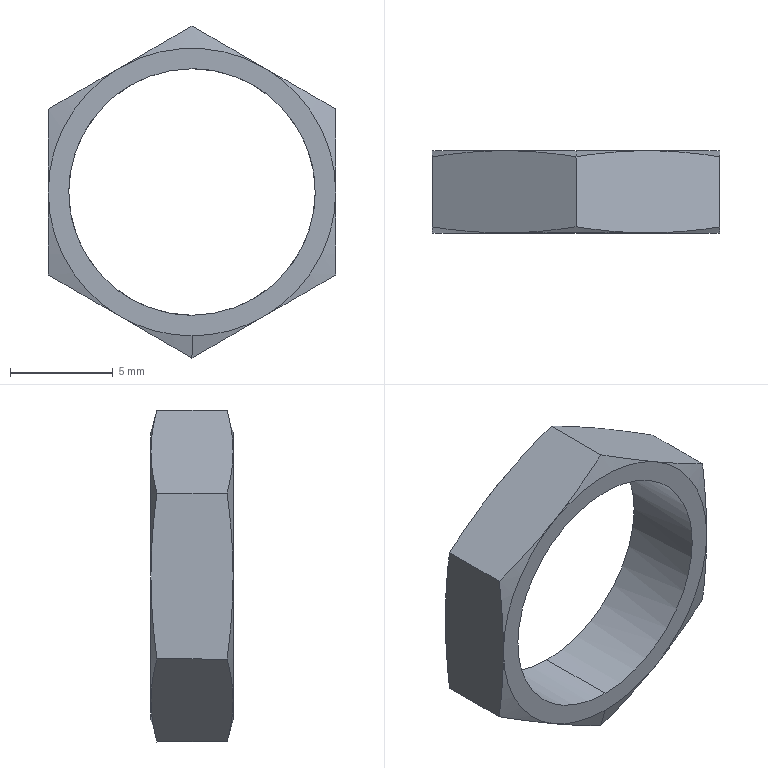Component | SolidWorks | HandlingMechanism-2_MVPTN2-1_4_1-1 | 1 solid | 24 faces | box 14 x 4 x 16.17 mm | volume 224 mm3 | cone 14 | plane 8 | cylinder 2 | commonest cylinder face diameters 12 x2
STEP:
#1=COLOUR_RGB('',0.7922,0.8196,0.9333);
#2=FILL_AREA_STYLE_COLOUR('',#1);
#3=FILL_AREA_STYLE('',(#2));
#4=SURFACE_STYLE_FILL_AREA(#3);
#5=SURFACE_SIDE_STYLE('',(#4));
#6=SURFACE_STYLE_USAGE(.BOTH.,#5);
#7=PRESENTATION_STYLE_ASSIGNMENT((#6));
#8=CARTESIAN_POINT('',(1.019,8.76,5.236));
#9=VERTEX_POINT('',#8);
#10=CARTESIAN_POINT('',(1.019,8.76,5.709));
#11=VERTEX_POINT('',#10);
#12=CARTESIAN_POINT('',(1.019,8.76,5.472));
#13=DIRECTION('',(-0.,-1.,0.));
#14=DIRECTION('',(0.,0.,1.));
#15=AXIS2_PLACEMENT_3D('',#12,#13,#14);
#16=CIRCLE('',#15,0.2362);
#17=EDGE_CURVE('',#9,#11,#16,.T.);
#18=ORIENTED_EDGE('',*,*,#17,.F.);
#19=CARTESIAN_POINT('',(1.019,8.602,5.236));
#20=VERTEX_POINT('',#19);
#21=CARTESIAN_POINT('',(1.019,8.76,5.236));
#22=DIRECTION('',(-0.,-1.,0.));
#23=VECTOR('',#22,39.37);
#24=LINE('',#21,#23);
#25=EDGE_CURVE('',#9,#20,#24,.T.);
#26=ORIENTED_EDGE('',*,*,#25,.T.);
#27=CARTESIAN_POINT('',(1.019,8.602,5.709));
#28=VERTEX_POINT('',#27);
#29=CARTESIAN_POINT('',(1.019,8.602,5.236));
#30=CARTESIAN_POINT('',(1.05,8.602,5.236));
#31=CARTESIAN_POINT('',(1.081,8.602,5.242));
#32=CARTESIAN_POINT('',(1.138,8.602,5.266));
#33=CARTESIAN_POINT('',(1.164,8.602,5.284));
#34=CARTESIAN_POINT('',(1.208,8.602,5.327));
#35=CARTESIAN_POINT('',(1.225,8.602,5.353));
#36=CARTESIAN_POINT('',(1.249,8.602,5.411));
#37=CARTESIAN_POINT('',(1.255,8.602,5.442));
#38=CARTESIAN_POINT('',(1.255,8.602,5.503));
#39=CARTESIAN_POINT('',(1.249,8.602,5.534));
#40=CARTESIAN_POINT('',(1.225,8.602,5.591));
#41=CARTESIAN_POINT('',(1.208,8.602,5.618));
#42=CARTESIAN_POINT('',(1.164,8.602,5.661));
#43=CARTESIAN_POINT('',(1.138,8.602,5.679));
#44=CARTESIAN_POINT('',(1.081,8.602,5.703));
#45=CARTESIAN_POINT('',(1.05,8.602,5.709));
#46=CARTESIAN_POINT('',(1.019,8.602,5.709));
#47=B_SPLINE_CURVE_WITH_KNOTS('',3,(#29,#30,#31,#32,#33,#34,#35,#36,#37,#38,#39,#40,#41,#42,#43,#44,#45,#46),.UNSPECIFIED.,.F.,.F.,(4,2,2,2,2,2,2,2,4),(0.5,0.5625,0.625,0.6875,0.75,0.8125,0.875,0.9375,1.),.UNSPECIFIED.);
#48=EDGE_CURVE('',#20,#28,#47,.T.);
#49=ORIENTED_EDGE('',*,*,#48,.T.);
#50=CARTESIAN_POINT('',(1.019,8.76,5.709));
#51=DIRECTION('',(-0.,-1.,0.));
#52=VECTOR('',#51,39.37);
#53=LINE('',#50,#52);
#54=EDGE_CURVE('',#11,#28,#53,.T.);
#55=ORIENTED_EDGE('',*,*,#54,.F.);
#56=EDGE_LOOP('',(#18,#26,#49,#55));
#57=FACE_OUTER_BOUND('',#56,.T.);
#58=CARTESIAN_POINT('',(1.019,8.76,5.472));
#59=DIRECTION('',(-0.,-1.,0.));
#60=DIRECTION('',(0.,0.,1.));
#61=AXIS2_PLACEMENT_3D('',#58,#59,#60);
#62=CYLINDRICAL_SURFACE('',#61,0.2362);
#63=ADVANCED_FACE('',(#57),#62,.F.);
#64=CARTESIAN_POINT('',(1.019,8.76,5.748));
#65=VERTEX_POINT('',#64);
#66=CARTESIAN_POINT('',(1.157,8.76,5.711));
#67=VERTEX_POINT('',#66);
#68=CARTESIAN_POINT('',(1.019,8.76,5.472));
#69=DIRECTION('',(0.,1.,-0.));
#70=DIRECTION('',(0.,0.,1.));
#71=AXIS2_PLACEMENT_3D('',#68,#69,#70);
#72=CIRCLE('',#71,0.2756);
#73=EDGE_CURVE('',#65,#67,#72,.T.);
#74=ORIENTED_EDGE('',*,*,#73,.F.);
#75=CARTESIAN_POINT('',(1.019,8.748,5.791));
#76=VERTEX_POINT('',#75);
#77=CARTESIAN_POINT('',(1.019,8.748,5.791));
#78=DIRECTION('',(-0.,-0.2588,0.9659));
#79=VECTOR('',#78,39.37);
#80=LINE('',#77,#79);
#81=EDGE_CURVE('',#65,#76,#80,.T.);
#82=ORIENTED_EDGE('',*,*,#81,.T.);
#83=CARTESIAN_POINT('',(1.019,8.748,5.791));
#84=CARTESIAN_POINT('',(1.065,8.755,5.764));
#85=CARTESIAN_POINT('',(1.111,8.76,5.738));
#86=CARTESIAN_POINT('',(1.157,8.76,5.711));
#87=B_SPLINE_CURVE_WITH_KNOTS('',3,(#83,#84,#85,#86),.UNSPECIFIED.,.F.,.F.,(4,4),(0.,0.004052),.UNSPECIFIED.);
#88=EDGE_CURVE('',#76,#67,#87,.T.);
#89=ORIENTED_EDGE('',*,*,#88,.T.);
#90=EDGE_LOOP('',(#74,#82,#89));
#91=FACE_OUTER_BOUND('',#90,.T.);
#92=CARTESIAN_POINT('',(1.019,8.748,5.472));
#93=DIRECTION('',(-0.,-1.,0.));
#94=DIRECTION('',(0.,0.,1.));
#95=AXIS2_PLACEMENT_3D('',#92,#93,#94);
#96=CONICAL_SURFACE('',#95,0.3185,1.309);
#97=ADVANCED_FACE('',(#91),#96,.T.);
#98=CARTESIAN_POINT('',(1.019,8.602,5.197));
#99=VERTEX_POINT('',#98);
#100=CARTESIAN_POINT('',(1.157,8.602,5.234));
#101=VERTEX_POINT('',#100);
#102=CARTESIAN_POINT('',(1.019,8.602,5.472));
#103=DIRECTION('',(-0.,-1.,0.));
#104=DIRECTION('',(0.,0.,-1.));
#105=AXIS2_PLACEMENT_3D('',#102,#103,#104);
#106=CIRCLE('',#105,0.2756);
#107=EDGE_CURVE('',#99,#101,#106,.T.);
#108=ORIENTED_EDGE('',*,*,#107,.F.);
#109=CARTESIAN_POINT('',(1.019,8.614,5.154));
#110=VERTEX_POINT('',#109);
#111=CARTESIAN_POINT('',(1.019,8.614,5.154));
#112=DIRECTION('',(0.,0.2588,-0.9659));
#113=VECTOR('',#112,39.37);
#114=LINE('',#111,#113);
#115=EDGE_CURVE('',#99,#110,#114,.T.);
#116=ORIENTED_EDGE('',*,*,#115,.T.);
#117=CARTESIAN_POINT('',(1.019,8.614,5.154));
#118=CARTESIAN_POINT('',(1.065,8.607,5.181));
#119=CARTESIAN_POINT('',(1.111,8.602,5.207));
#120=CARTESIAN_POINT('',(1.157,8.602,5.234));
#121=B_SPLINE_CURVE_WITH_KNOTS('',3,(#117,#118,#119,#120),.UNSPECIFIED.,.F.,.F.,(4,4),(0.,0.004052),.UNSPECIFIED.);
#122=EDGE_CURVE('',#110,#101,#121,.T.);
#123=ORIENTED_EDGE('',*,*,#122,.T.);
#124=EDGE_LOOP('',(#108,#116,#123));
#125=FACE_OUTER_BOUND('',#124,.T.);
#126=CARTESIAN_POINT('',(1.019,8.614,5.472));
#127=DIRECTION('',(0.,1.,-0.));
#128=DIRECTION('',(0.,0.,-1.));
#129=AXIS2_PLACEMENT_3D('',#126,#127,#128);
#130=CONICAL_SURFACE('',#129,0.3185,1.309);
#131=ADVANCED_FACE('',(#125),#130,.T.);
#132=CARTESIAN_POINT('',(1.157,8.76,5.234));
#133=VERTEX_POINT('',#132);
#134=CARTESIAN_POINT('',(0.8811,8.76,5.234));
#135=VERTEX_POINT('',#134);
#136=CARTESIAN_POINT('',(1.019,8.76,5.472));
#137=DIRECTION('',(0.,1.,-0.));
#138=DIRECTION('',(-0.,0.,1.));
#139=AXIS2_PLACEMENT_3D('',#136,#137,#138);
#140=CIRCLE('',#139,0.2756);
#141=EDGE_CURVE('',#133,#135,#140,.T.);
#142=ORIENTED_EDGE('',*,*,#141,.T.);
#143=CARTESIAN_POINT('',(0.7433,8.76,5.472));
#144=VERTEX_POINT('',#143);
#145=CARTESIAN_POINT('',(1.019,8.76,5.472));
#146=DIRECTION('',(0.,1.,-0.));
#147=DIRECTION('',(0.,0.,1.));
#148=AXIS2_PLACEMENT_3D('',#145,#146,#147);
#149=CIRCLE('',#148,0.2756);
#150=EDGE_CURVE('',#135,#144,#149,.T.);
#151=ORIENTED_EDGE('',*,*,#150,.T.);
#152=CARTESIAN_POINT('',(0.8811,8.76,5.711));
#153=VERTEX_POINT('',#152);
#154=CARTESIAN_POINT('',(1.019,8.76,5.472));
#155=DIRECTION('',(0.,1.,-0.));
#156=DIRECTION('',(0.,0.,1.));
#157=AXIS2_PLACEMENT_3D('',#154,#155,#156);
#158=CIRCLE('',#157,0.2756);
#159=EDGE_CURVE('',#144,#153,#158,.T.);
#160=ORIENTED_EDGE('',*,*,#159,.T.);
#161=CARTESIAN_POINT('',(1.019,8.76,5.472));
#162=DIRECTION('',(0.,1.,-0.));
#163=DIRECTION('',(-0.,0.,1.));
#164=AXIS2_PLACEMENT_3D('',#161,#162,#163);
#165=CIRCLE('',#164,0.2756);
#166=EDGE_CURVE('',#153,#65,#165,.T.);
#167=ORIENTED_EDGE('',*,*,#166,.T.);
#168=ORIENTED_EDGE('',*,*,#73,.T.);
#169=CARTESIAN_POINT('',(1.295,8.76,5.472));
#170=VERTEX_POINT('',#169);
#171=CARTESIAN_POINT('',(1.019,8.76,5.472));
#172=DIRECTION('',(0.,1.,-0.));
#173=DIRECTION('',(0.,0.,1.));
#174=AXIS2_PLACEMENT_3D('',#171,#172,#173);
#175=CIRCLE('',#174,0.2756);
#176=EDGE_CURVE('',#67,#170,#175,.T.);
#177=ORIENTED_EDGE('',*,*,#176,.T.);
#178=CARTESIAN_POINT('',(1.019,8.76,5.472));
#179=DIRECTION('',(0.,1.,-0.));
#180=DIRECTION('',(0.,0.,1.));
#181=AXIS2_PLACEMENT_3D('',#178,#179,#180);
#182=CIRCLE('',#181,0.2756);
#183=EDGE_CURVE('',#170,#133,#182,.T.);
#184=ORIENTED_EDGE('',*,*,#183,.T.);
#185=EDGE_LOOP('',(#142,#151,#160,#167,#168,#177,#184));
#186=FACE_OUTER_BOUND('',#185,.T.);
#187=CARTESIAN_POINT('',(1.019,8.76,5.472));
#188=DIRECTION('',(-0.,-1.,0.));
#189=DIRECTION('',(0.,0.,1.));
#190=AXIS2_PLACEMENT_3D('',#187,#188,#189);
#191=CIRCLE('',#190,0.2362);
#192=EDGE_CURVE('',#11,#9,#191,.T.);
#193=ORIENTED_EDGE('',*,*,#192,.T.);
#194=ORIENTED_EDGE('',*,*,#17,.T.);
#195=EDGE_LOOP('',(#193,#194));
#196=FACE_BOUND('',#195,.T.);
#197=CARTESIAN_POINT('',(0.8811,8.76,5.472));
#198=DIRECTION('',(0.,1.,-0.));
#199=DIRECTION('',(0.,-0.,-1.));
#200=AXIS2_PLACEMENT_3D('',#197,#198,#199);
#201=PLANE('',#200);
#202=ADVANCED_FACE('',(#186,#196),#201,.T.);
#203=CARTESIAN_POINT('',(1.295,8.602,5.472));
#204=VERTEX_POINT('',#203);
#205=CARTESIAN_POINT('',(1.157,8.602,5.711));
#206=VERTEX_POINT('',#205);
#207=CARTESIAN_POINT('',(1.019,8.602,5.472));
#208=DIRECTION('',(-0.,-1.,0.));
#209=DIRECTION('',(0.,0.,-1.));
#210=AXIS2_PLACEMENT_3D('',#207,#208,#209);
#211=CIRCLE('',#210,0.2756);
#212=EDGE_CURVE('',#204,#206,#211,.T.);
#213=ORIENTED_EDGE('',*,*,#212,.T.);
#214=CARTESIAN_POINT('',(0.8811,8.602,5.711));
#215=VERTEX_POINT('',#214);
#216=CARTESIAN_POINT('',(1.019,8.602,5.472));
#217=DIRECTION('',(-0.,-1.,0.));
#218=DIRECTION('',(-0.,0.,-1.));
#219=AXIS2_PLACEMENT_3D('',#216,#217,#218);
#220=CIRCLE('',#219,0.2756);
#221=EDGE_CURVE('',#206,#215,#220,.T.);
#222=ORIENTED_EDGE('',*,*,#221,.T.);
#223=CARTESIAN_POINT('',(0.7433,8.602,5.472));
#224=VERTEX_POINT('',#223);
#225=CARTESIAN_POINT('',(1.019,8.602,5.472));
#226=DIRECTION('',(-0.,-1.,0.));
#227=DIRECTION('',(0.,0.,-1.));
#228=AXIS2_PLACEMENT_3D('',#225,#226,#227);
#229=CIRCLE('',#228,0.2756);
#230=EDGE_CURVE('',#215,#224,#229,.T.);
#231=ORIENTED_EDGE('',*,*,#230,.T.);
#232=CARTESIAN_POINT('',(0.8811,8.602,5.234));
#233=VERTEX_POINT('',#232);
#234=CARTESIAN_POINT('',(1.019,8.602,5.472));
#235=DIRECTION('',(-0.,-1.,0.));
#236=DIRECTION('',(0.,0.,-1.));
#237=AXIS2_PLACEMENT_3D('',#234,#235,#236);
#238=CIRCLE('',#237,0.2756);
#239=EDGE_CURVE('',#224,#233,#238,.T.);
#240=ORIENTED_EDGE('',*,*,#239,.T.);
#241=CARTESIAN_POINT('',(1.019,8.602,5.472));
#242=DIRECTION('',(-0.,-1.,0.));
#243=DIRECTION('',(-0.,0.,-1.));
#244=AXIS2_PLACEMENT_3D('',#241,#242,#243);
#245=CIRCLE('',#244,0.2756);
#246=EDGE_CURVE('',#233,#99,#245,.T.);
#247=ORIENTED_EDGE('',*,*,#246,.T.);
#248=ORIENTED_EDGE('',*,*,#107,.T.);
#249=CARTESIAN_POINT('',(1.019,8.602,5.472));
#250=DIRECTION('',(-0.,-1.,0.));
#251=DIRECTION('',(0.,0.,-1.));
#252=AXIS2_PLACEMENT_3D('',#249,#250,#251);
#253=CIRCLE('',#252,0.2756);
#254=EDGE_CURVE('',#101,#204,#253,.T.);
#255=ORIENTED_EDGE('',*,*,#254,.T.);
#256=EDGE_LOOP('',(#213,#222,#231,#240,#247,#248,#255));
#257=FACE_OUTER_BOUND('',#256,.T.);
#258=CARTESIAN_POINT('',(1.019,8.602,5.709));
#259=CARTESIAN_POINT('',(0.988,8.602,5.709));
#260=CARTESIAN_POINT('',(0.9571,8.602,5.703));
#261=CARTESIAN_POINT('',(0.9,8.602,5.679));
#262=CARTESIAN_POINT('',(0.8738,8.602,5.661));
#263=CARTESIAN_POINT('',(0.83,8.602,5.618));
#264=CARTESIAN_POINT('',(0.8125,8.602,5.591));
#265=CARTESIAN_POINT('',(0.7888,8.602,5.534));
#266=CARTESIAN_POINT('',(0.7827,8.602,5.503));
#267=CARTESIAN_POINT('',(0.7827,8.602,5.442));
#268=CARTESIAN_POINT('',(0.7888,8.602,5.411));
#269=CARTESIAN_POINT('',(0.8125,8.602,5.353));
#270=CARTESIAN_POINT('',(0.83,8.602,5.327));
#271=CARTESIAN_POINT('',(0.8738,8.602,5.284));
#272=CARTESIAN_POINT('',(0.9,8.602,5.266));
#273=CARTESIAN_POINT('',(0.9571,8.602,5.242));
#274=CARTESIAN_POINT('',(0.988,8.602,5.236));
#275=CARTESIAN_POINT('',(1.019,8.602,5.236));
#276=B_SPLINE_CURVE_WITH_KNOTS('',3,(#258,#259,#260,#261,#262,#263,#264,#265,#266,#267,#268,#269,#270,#271,#272,#273,#274,#275),.UNSPECIFIED.,.F.,.F.,(4,2,2,2,2,2,2,2,4),(0.,0.0625,0.125,0.1875,0.25,0.3125,0.375,0.4375,0.5),.UNSPECIFIED.);
#277=EDGE_CURVE('',#28,#20,#276,.T.);
#278=ORIENTED_EDGE('',*,*,#277,.F.);
#279=ORIENTED_EDGE('',*,*,#48,.F.);
#280=EDGE_LOOP('',(#278,#279));
#281=FACE_BOUND('',#280,.T.);
#282=CARTESIAN_POINT('',(0.8811,8.602,5.472));
#283=DIRECTION('',(-0.,-1.,0.));
#284=DIRECTION('',(-0.,0.,1.));
#285=AXIS2_PLACEMENT_3D('',#282,#283,#284);
#286=PLANE('',#285);
#287=ADVANCED_FACE('',(#257,#281),#286,.T.);
#288=ORIENTED_EDGE('',*,*,#150,.F.);
#289=CARTESIAN_POINT('',(0.7433,8.748,5.313));
#290=VERTEX_POINT('',#289);
#291=CARTESIAN_POINT('',(0.8811,8.76,5.234));
#292=CARTESIAN_POINT('',(0.835,8.76,5.26));
#293=CARTESIAN_POINT('',(0.7891,8.755,5.287));
#294=CARTESIAN_POINT('',(0.7433,8.748,5.313));
#295=B_SPLINE_CURVE_WITH_KNOTS('',3,(#291,#292,#293,#294),.UNSPECIFIED.,.F.,.F.,(4,4),(0.,0.004052),.UNSPECIFIED.);
#296=EDGE_CURVE('',#135,#290,#295,.T.);
#297=ORIENTED_EDGE('',*,*,#296,.T.);
#298=CARTESIAN_POINT('',(0.7433,8.748,5.313));
#299=CARTESIAN_POINT('',(0.7433,8.755,5.366));
#300=CARTESIAN_POINT('',(0.7433,8.76,5.419));
#301=CARTESIAN_POINT('',(0.7433,8.76,5.472));
#302=B_SPLINE_CURVE_WITH_KNOTS('',3,(#298,#299,#300,#301),.UNSPECIFIED.,.F.,.F.,(4,4),(0.,0.004052),.UNSPECIFIED.);
#303=EDGE_CURVE('',#290,#144,#302,.T.);
#304=ORIENTED_EDGE('',*,*,#303,.T.);
#305=EDGE_LOOP('',(#288,#297,#304));
#306=FACE_OUTER_BOUND('',#305,.T.);
#307=CARTESIAN_POINT('',(1.019,8.748,5.472));
#308=DIRECTION('',(-0.,-1.,0.));
#309=DIRECTION('',(0.,0.,1.));
#310=AXIS2_PLACEMENT_3D('',#307,#308,#309);
#311=CONICAL_SURFACE('',#310,0.3185,1.309);
#312=ADVANCED_FACE('',(#306),#311,.T.);
#313=ORIENTED_EDGE('',*,*,#141,.F.);
#314=CARTESIAN_POINT('',(1.019,8.748,5.154));
#315=VERTEX_POINT('',#314);
#316=CARTESIAN_POINT('',(1.157,8.76,5.234));
#317=CARTESIAN_POINT('',(1.111,8.76,5.207));
#318=CARTESIAN_POINT('',(1.065,8.755,5.181));
#319=CARTESIAN_POINT('',(1.019,8.748,5.154));
#320=B_SPLINE_CURVE_WITH_KNOTS('',3,(#316,#317,#318,#319),.UNSPECIFIED.,.F.,.F.,(4,4),(0.,0.004052),.UNSPECIFIED.);
#321=EDGE_CURVE('',#133,#315,#320,.T.);
#322=ORIENTED_EDGE('',*,*,#321,.T.);
#323=CARTESIAN_POINT('',(1.019,8.748,5.154));
#324=CARTESIAN_POINT('',(0.9732,8.755,5.181));
#325=CARTESIAN_POINT('',(0.9273,8.76,5.207));
#326=CARTESIAN_POINT('',(0.8811,8.76,5.234));
#327=B_SPLINE_CURVE_WITH_KNOTS('',3,(#323,#324,#325,#326),.UNSPECIFIED.,.F.,.F.,(4,4),(0.,0.004052),.UNSPECIFIED.);
#328=EDGE_CURVE('',#315,#135,#327,.T.);
#329=ORIENTED_EDGE('',*,*,#328,.T.);
#330=EDGE_LOOP('',(#313,#322,#329));
#331=FACE_OUTER_BOUND('',#330,.T.);
#332=CARTESIAN_POINT('',(1.019,8.748,5.472));
#333=DIRECTION('',(-0.,-1.,0.));
#334=DIRECTION('',(0.,0.,1.));
#335=AXIS2_PLACEMENT_3D('',#332,#333,#334);
#336=CONICAL_SURFACE('',#335,0.3185,1.309);
#337=ADVANCED_FACE('',(#331),#336,.T.);
#338=ORIENTED_EDGE('',*,*,#183,.F.);
#339=CARTESIAN_POINT('',(1.295,8.748,5.313));
#340=VERTEX_POINT('',#339);
#341=CARTESIAN_POINT('',(1.295,8.76,5.472));
#342=CARTESIAN_POINT('',(1.295,8.76,5.419));
#343=CARTESIAN_POINT('',(1.295,8.755,5.366));
#344=CARTESIAN_POINT('',(1.295,8.748,5.313));
#345=B_SPLINE_CURVE_WITH_KNOTS('',3,(#341,#342,#343,#344),.UNSPECIFIED.,.F.,.F.,(4,4),(0.,0.004052),.UNSPECIFIED.);
#346=EDGE_CURVE('',#170,#340,#345,.T.);
#347=ORIENTED_EDGE('',*,*,#346,.T.);
#348=CARTESIAN_POINT('',(1.295,8.748,5.313));
#349=CARTESIAN_POINT('',(1.249,8.755,5.287));
#350=CARTESIAN_POINT('',(1.203,8.76,5.26));
#351=CARTESIAN_POINT('',(1.157,8.76,5.234));
#352=B_SPLINE_CURVE_WITH_KNOTS('',3,(#348,#349,#350,#351),.UNSPECIFIED.,.F.,.F.,(4,4),(0.,0.004052),.UNSPECIFIED.);
#353=EDGE_CURVE('',#340,#133,#352,.T.);
#354=ORIENTED_EDGE('',*,*,#353,.T.);
#355=EDGE_LOOP('',(#338,#347,#354));
#356=FACE_OUTER_BOUND('',#355,.T.);
#357=CARTESIAN_POINT('',(1.019,8.748,5.472));
#358=DIRECTION('',(-0.,-1.,0.));
#359=DIRECTION('',(0.,0.,1.));
#360=AXIS2_PLACEMENT_3D('',#357,#358,#359);
#361=CONICAL_SURFACE('',#360,0.3185,1.309);
#362=ADVANCED_FACE('',(#356),#361,.T.);
#363=CARTESIAN_POINT('',(1.295,8.748,5.632));
#364=VERTEX_POINT('',#363);
#365=CARTESIAN_POINT('',(1.295,8.748,5.632));
#366=CARTESIAN_POINT('',(1.295,8.755,5.579));
#367=CARTESIAN_POINT('',(1.295,8.76,5.526));
#368=CARTESIAN_POINT('',(1.295,8.76,5.472));
#369=B_SPLINE_CURVE_WITH_KNOTS('',3,(#365,#366,#367,#368),.UNSPECIFIED.,.F.,.F.,(4,4),(0.,0.004052),.UNSPECIFIED.);
#370=EDGE_CURVE('',#364,#170,#369,.T.);
#371=ORIENTED_EDGE('',*,*,#370,.T.);
#372=ORIENTED_EDGE('',*,*,#176,.F.);
#373=CARTESIAN_POINT('',(1.157,8.76,5.711));
#374=CARTESIAN_POINT('',(1.203,8.76,5.684));
#375=CARTESIAN_POINT('',(1.249,8.755,5.658));
#376=CARTESIAN_POINT('',(1.295,8.748,5.632));
#377=B_SPLINE_CURVE_WITH_KNOTS('',3,(#373,#374,#375,#376),.UNSPECIFIED.,.F.,.F.,(4,4),(0.,0.004052),.UNSPECIFIED.);
#378=EDGE_CURVE('',#67,#364,#377,.T.);
#379=ORIENTED_EDGE('',*,*,#378,.T.);
#380=EDGE_LOOP('',(#371,#372,#379));
#381=FACE_OUTER_BOUND('',#380,.T.);
#382=CARTESIAN_POINT('',(1.019,8.748,5.472));
#383=DIRECTION('',(-0.,-1.,0.));
#384=DIRECTION('',(0.,0.,1.));
#385=AXIS2_PLACEMENT_3D('',#382,#383,#384);
#386=CONICAL_SURFACE('',#385,0.3185,1.309);
#387=ADVANCED_FACE('',(#381),#386,.T.);
#388=ORIENTED_EDGE('',*,*,#81,.F.);
#389=ORIENTED_EDGE('',*,*,#166,.F.);
#390=CARTESIAN_POINT('',(0.8811,8.76,5.711));
#391=CARTESIAN_POINT('',(0.9273,8.76,5.738));
#392=CARTESIAN_POINT('',(0.9732,8.755,5.764));
#393=CARTESIAN_POINT('',(1.019,8.748,5.791));
#394=B_SPLINE_CURVE_WITH_KNOTS('',3,(#390,#391,#392,#393),.UNSPECIFIED.,.F.,.F.,(4,4),(0.,0.004052),.UNSPECIFIED.);
#395=EDGE_CURVE('',#153,#76,#394,.T.);
#396=ORIENTED_EDGE('',*,*,#395,.T.);
#397=EDGE_LOOP('',(#388,#389,#396));
#398=FACE_OUTER_BOUND('',#397,.T.);
#399=CARTESIAN_POINT('',(1.019,8.748,5.472));
#400=DIRECTION('',(-0.,-1.,0.));
#401=DIRECTION('',(0.,0.,1.));
#402=AXIS2_PLACEMENT_3D('',#399,#400,#401);
#403=CONICAL_SURFACE('',#402,0.3185,1.309);
#404=ADVANCED_FACE('',(#398),#403,.T.);
#405=CARTESIAN_POINT('',(0.7433,8.748,5.632));
#406=VERTEX_POINT('',#405);
#407=CARTESIAN_POINT('',(0.7433,8.748,5.632));
#408=CARTESIAN_POINT('',(0.7891,8.755,5.658));
#409=CARTESIAN_POINT('',(0.835,8.76,5.684));
#410=CARTESIAN_POINT('',(0.8811,8.76,5.711));
#411=B_SPLINE_CURVE_WITH_KNOTS('',3,(#407,#408,#409,#410),.UNSPECIFIED.,.F.,.F.,(4,4),(0.,0.004052),.UNSPECIFIED.);
#412=EDGE_CURVE('',#406,#153,#411,.T.);
#413=ORIENTED_EDGE('',*,*,#412,.T.);
#414=ORIENTED_EDGE('',*,*,#159,.F.);
#415=CARTESIAN_POINT('',(0.7433,8.76,5.472));
#416=CARTESIAN_POINT('',(0.7433,8.76,5.526));
#417=CARTESIAN_POINT('',(0.7433,8.755,5.579));
#418=CARTESIAN_POINT('',(0.7433,8.748,5.632));
#419=B_SPLINE_CURVE_WITH_KNOTS('',3,(#415,#416,#417,#418),.UNSPECIFIED.,.F.,.F.,(4,4),(0.,0.004052),.UNSPECIFIED.);
#420=EDGE_CURVE('',#144,#406,#419,.T.);
#421=ORIENTED_EDGE('',*,*,#420,.T.);
#422=EDGE_LOOP('',(#413,#414,#421));
#423=FACE_OUTER_BOUND('',#422,.T.);
#424=CARTESIAN_POINT('',(1.019,8.748,5.472));
#425=DIRECTION('',(-0.,-1.,0.));
#426=DIRECTION('',(0.,0.,1.));
#427=AXIS2_PLACEMENT_3D('',#424,#425,#426);
#428=CONICAL_SURFACE('',#427,0.3185,1.309);
#429=ADVANCED_FACE('',(#423),#428,.T.);
#430=CARTESIAN_POINT('',(1.019,8.614,5.791));
#431=VERTEX_POINT('',#430);
#432=CARTESIAN_POINT('',(1.019,8.614,5.791));
#433=CARTESIAN_POINT('',(0.9732,8.607,5.764));
#434=CARTESIAN_POINT('',(0.9273,8.602,5.738));
#435=CARTESIAN_POINT('',(0.8811,8.602,5.711));
#436=B_SPLINE_CURVE_WITH_KNOTS('',3,(#432,#433,#434,#435),.UNSPECIFIED.,.F.,.F.,(4,4),(0.,0.004052),.UNSPECIFIED.);
#437=EDGE_CURVE('',#431,#215,#436,.T.);
#438=ORIENTED_EDGE('',*,*,#437,.T.);
#439=ORIENTED_EDGE('',*,*,#221,.F.);
#440=CARTESIAN_POINT('',(1.157,8.602,5.711));
#441=CARTESIAN_POINT('',(1.111,8.602,5.738));
#442=CARTESIAN_POINT('',(1.065,8.607,5.764));
#443=CARTESIAN_POINT('',(1.019,8.614,5.791));
#444=B_SPLINE_CURVE_WITH_KNOTS('',3,(#440,#441,#442,#443),.UNSPECIFIED.,.F.,.F.,(4,4),(0.,0.004052),.UNSPECIFIED.);
#445=EDGE_CURVE('',#206,#431,#444,.T.);
#446=ORIENTED_EDGE('',*,*,#445,.T.);
#447=EDGE_LOOP('',(#438,#439,#446));
#448=FACE_OUTER_BOUND('',#447,.T.);
#449=CARTESIAN_POINT('',(1.019,8.614,5.472));
#450=DIRECTION('',(0.,1.,-0.));
#451=DIRECTION('',(0.,0.,-1.));
#452=AXIS2_PLACEMENT_3D('',#449,#450,#451);
#453=CONICAL_SURFACE('',#452,0.3185,1.309);
#454=ADVANCED_FACE('',(#448),#453,.T.);
#455=CARTESIAN_POINT('',(1.295,8.614,5.632));
#456=VERTEX_POINT('',#455);
#457=CARTESIAN_POINT('',(1.295,8.614,5.632));
#458=CARTESIAN_POINT('',(1.249,8.607,5.658));
#459=CARTESIAN_POINT('',(1.203,8.602,5.684));
#460=CARTESIAN_POINT('',(1.157,8.602,5.711));
#461=B_SPLINE_CURVE_WITH_KNOTS('',3,(#457,#458,#459,#460),.UNSPECIFIED.,.F.,.F.,(4,4),(0.,0.004052),.UNSPECIFIED.);
#462=EDGE_CURVE('',#456,#206,#461,.T.);
#463=ORIENTED_EDGE('',*,*,#462,.T.);
#464=ORIENTED_EDGE('',*,*,#212,.F.);
#465=CARTESIAN_POINT('',(1.295,8.602,5.472));
#466=CARTESIAN_POINT('',(1.295,8.602,5.526));
#467=CARTESIAN_POINT('',(1.295,8.607,5.579));
#468=CARTESIAN_POINT('',(1.295,8.614,5.632));
#469=B_SPLINE_CURVE_WITH_KNOTS('',3,(#465,#466,#467,#468),.UNSPECIFIED.,.F.,.F.,(4,4),(0.,0.004052),.UNSPECIFIED.);
#470=EDGE_CURVE('',#204,#456,#469,.T.);
#471=ORIENTED_EDGE('',*,*,#470,.T.);
#472=EDGE_LOOP('',(#463,#464,#471));
#473=FACE_OUTER_BOUND('',#472,.T.);
#474=CARTESIAN_POINT('',(1.019,8.614,5.472));
#475=DIRECTION('',(0.,1.,-0.));
#476=DIRECTION('',(0.,0.,-1.));
#477=AXIS2_PLACEMENT_3D('',#474,#475,#476);
#478=CONICAL_SURFACE('',#477,0.3185,1.309);
#479=ADVANCED_FACE('',(#473),#478,.T.);
#480=CARTESIAN_POINT('',(1.295,8.614,5.313));
#481=VERTEX_POINT('',#480);
#482=CARTESIAN_POINT('',(1.295,8.614,5.313));
#483=CARTESIAN_POINT('',(1.295,8.607,5.366));
#484=CARTESIAN_POINT('',(1.295,8.602,5.419));
#485=CARTESIAN_POINT('',(1.295,8.602,5.472));
#486=B_SPLINE_CURVE_WITH_KNOTS('',3,(#482,#483,#484,#485),.UNSPECIFIED.,.F.,.F.,(4,4),(0.,0.004052),.UNSPECIFIED.);
#487=EDGE_CURVE('',#481,#204,#486,.T.);
#488=ORIENTED_EDGE('',*,*,#487,.T.);
#489=ORIENTED_EDGE('',*,*,#254,.F.);
#490=CARTESIAN_POINT('',(1.157,8.602,5.234));
#491=CARTESIAN_POINT('',(1.203,8.602,5.26));
#492=CARTESIAN_POINT('',(1.249,8.607,5.287));
#493=CARTESIAN_POINT('',(1.295,8.614,5.313));
#494=B_SPLINE_CURVE_WITH_KNOTS('',3,(#490,#491,#492,#493),.UNSPECIFIED.,.F.,.F.,(4,4),(0.,0.004052),.UNSPECIFIED.);
#495=EDGE_CURVE('',#101,#481,#494,.T.);
#496=ORIENTED_EDGE('',*,*,#495,.T.);
#497=EDGE_LOOP('',(#488,#489,#496));
#498=FACE_OUTER_BOUND('',#497,.T.);
#499=CARTESIAN_POINT('',(1.019,8.614,5.472));
#500=DIRECTION('',(0.,1.,-0.));
#501=DIRECTION('',(0.,0.,-1.));
#502=AXIS2_PLACEMENT_3D('',#499,#500,#501);
#503=CONICAL_SURFACE('',#502,0.3185,1.309);
#504=ADVANCED_FACE('',(#498),#503,.T.);
#505=ORIENTED_EDGE('',*,*,#115,.F.);
#506=ORIENTED_EDGE('',*,*,#246,.F.);
#507=CARTESIAN_POINT('',(0.8811,8.602,5.234));
#508=CARTESIAN_POINT('',(0.9273,8.602,5.207));
#509=CARTESIAN_POINT('',(0.9732,8.607,5.181));
#510=CARTESIAN_POINT('',(1.019,8.614,5.154));
#511=B_SPLINE_CURVE_WITH_KNOTS('',3,(#507,#508,#509,#510),.UNSPECIFIED.,.F.,.F.,(4,4),(0.,0.004052),.UNSPECIFIED.);
#512=EDGE_CURVE('',#233,#110,#511,.T.);
#513=ORIENTED_EDGE('',*,*,#512,.T.);
#514=EDGE_LOOP('',(#505,#506,#513));
#515=FACE_OUTER_BOUND('',#514,.T.);
#516=CARTESIAN_POINT('',(1.019,8.614,5.472));
#517=DIRECTION('',(0.,1.,-0.));
#518=DIRECTION('',(0.,0.,-1.));
#519=AXIS2_PLACEMENT_3D('',#516,#517,#518);
#520=CONICAL_SURFACE('',#519,0.3185,1.309);
#521=ADVANCED_FACE('',(#515),#520,.T.);
#522=ORIENTED_EDGE('',*,*,#239,.F.);
#523=CARTESIAN_POINT('',(0.7433,8.614,5.313));
#524=VERTEX_POINT('',#523);
#525=CARTESIAN_POINT('',(0.7433,8.602,5.472));
#526=CARTESIAN_POINT('',(0.7433,8.602,5.419));
#527=CARTESIAN_POINT('',(0.7433,8.607,5.366));
#528=CARTESIAN_POINT('',(0.7433,8.614,5.313));
#529=B_SPLINE_CURVE_WITH_KNOTS('',3,(#525,#526,#527,#528),.UNSPECIFIED.,.F.,.F.,(4,4),(0.,0.004052),.UNSPECIFIED.);
#530=EDGE_CURVE('',#224,#524,#529,.T.);
#531=ORIENTED_EDGE('',*,*,#530,.T.);
#532=CARTESIAN_POINT('',(0.7433,8.614,5.313));
#533=CARTESIAN_POINT('',(0.7891,8.607,5.287));
#534=CARTESIAN_POINT('',(0.835,8.602,5.26));
#535=CARTESIAN_POINT('',(0.8811,8.602,5.234));
#536=B_SPLINE_CURVE_WITH_KNOTS('',3,(#532,#533,#534,#535),.UNSPECIFIED.,.F.,.F.,(4,4),(0.,0.004052),.UNSPECIFIED.);
#537=EDGE_CURVE('',#524,#233,#536,.T.);
#538=ORIENTED_EDGE('',*,*,#537,.T.);
#539=EDGE_LOOP('',(#522,#531,#538));
#540=FACE_OUTER_BOUND('',#539,.T.);
#541=CARTESIAN_POINT('',(1.019,8.614,5.472));
#542=DIRECTION('',(0.,1.,-0.));
#543=DIRECTION('',(0.,0.,-1.));
#544=AXIS2_PLACEMENT_3D('',#541,#542,#543);
#545=CONICAL_SURFACE('',#544,0.3185,1.309);
#546=ADVANCED_FACE('',(#540),#545,.T.);
#547=ORIENTED_EDGE('',*,*,#230,.F.);
#548=CARTESIAN_POINT('',(0.7433,8.614,5.632));
#549=VERTEX_POINT('',#548);
#550=CARTESIAN_POINT('',(0.8811,8.602,5.711));
#551=CARTESIAN_POINT('',(0.835,8.602,5.684));
#552=CARTESIAN_POINT('',(0.7891,8.607,5.658));
#553=CARTESIAN_POINT('',(0.7433,8.614,5.632));
#554=B_SPLINE_CURVE_WITH_KNOTS('',3,(#550,#551,#552,#553),.UNSPECIFIED.,.F.,.F.,(4,4),(0.,0.004052),.UNSPECIFIED.);
#555=EDGE_CURVE('',#215,#549,#554,.T.);
#556=ORIENTED_EDGE('',*,*,#555,.T.);
#557=CARTESIAN_POINT('',(0.7433,8.614,5.632));
#558=CARTESIAN_POINT('',(0.7433,8.607,5.579));
#559=CARTESIAN_POINT('',(0.7433,8.602,5.526));
#560=CARTESIAN_POINT('',(0.7433,8.602,5.472));
#561=B_SPLINE_CURVE_WITH_KNOTS('',3,(#557,#558,#559,#560),.UNSPECIFIED.,.F.,.F.,(4,4),(0.,0.004052),.UNSPECIFIED.);
#562=EDGE_CURVE('',#549,#224,#561,.T.);
#563=ORIENTED_EDGE('',*,*,#562,.T.);
#564=EDGE_LOOP('',(#547,#556,#563));
#565=FACE_OUTER_BOUND('',#564,.T.);
#566=CARTESIAN_POINT('',(1.019,8.614,5.472));
#567=DIRECTION('',(0.,1.,-0.));
#568=DIRECTION('',(0.,0.,-1.));
#569=AXIS2_PLACEMENT_3D('',#566,#567,#568);
#570=CONICAL_SURFACE('',#569,0.3185,1.309);
#571=ADVANCED_FACE('',(#565),#570,.T.);
#572=ORIENTED_EDGE('',*,*,#537,.F.);
#573=CARTESIAN_POINT('',(0.7433,8.76,5.313));
#574=DIRECTION('',(-0.,-1.,0.));
#575=VECTOR('',#574,39.37);
#576=LINE('',#573,#575);
#577=EDGE_CURVE('',#290,#524,#576,.T.);
#578=ORIENTED_EDGE('',*,*,#577,.F.);
#579=ORIENTED_EDGE('',*,*,#296,.F.);
#580=ORIENTED_EDGE('',*,*,#328,.F.);
#581=CARTESIAN_POINT('',(1.019,8.76,5.154));
#582=DIRECTION('',(0.,1.,-0.));
#583=VECTOR('',#582,39.37);
#584=LINE('',#581,#583);
#585=EDGE_CURVE('',#110,#315,#584,.T.);
#586=ORIENTED_EDGE('',*,*,#585,.F.);
#587=ORIENTED_EDGE('',*,*,#512,.F.);
#588=EDGE_LOOP('',(#572,#578,#579,#580,#586,#587));
#589=FACE_OUTER_BOUND('',#588,.T.);
#590=CARTESIAN_POINT('',(0.7433,8.76,5.313));
#591=DIRECTION('',(0.5,-0.,0.866));
#592=DIRECTION('',(-0.866,0.,0.5));
#593=AXIS2_PLACEMENT_3D('',#590,#591,#592);
#594=PLANE('',#593);
#595=ADVANCED_FACE('',(#589),#594,.F.);
#596=ORIENTED_EDGE('',*,*,#562,.F.);
#597=CARTESIAN_POINT('',(0.7433,8.76,5.632));
#598=DIRECTION('',(-0.,-1.,0.));
#599=VECTOR('',#598,39.37);
#600=LINE('',#597,#599);
#601=EDGE_CURVE('',#406,#549,#600,.T.);
#602=ORIENTED_EDGE('',*,*,#601,.F.);
#603=ORIENTED_EDGE('',*,*,#420,.F.);
#604=ORIENTED_EDGE('',*,*,#303,.F.);
#605=ORIENTED_EDGE('',*,*,#577,.T.);
#606=ORIENTED_EDGE('',*,*,#530,.F.);
#607=EDGE_LOOP('',(#596,#602,#603,#604,#605,#606));
#608=FACE_OUTER_BOUND('',#607,.T.);
#609=CARTESIAN_POINT('',(0.7433,8.76,5.632));
#610=DIRECTION('',(1.,-0.,0.));
#611=DIRECTION('',(-0.,0.,1.));
#612=AXIS2_PLACEMENT_3D('',#609,#610,#611);
#613=PLANE('',#612);
#614=ADVANCED_FACE('',(#608),#613,.F.);
#615=ORIENTED_EDGE('',*,*,#585,.T.);
#616=ORIENTED_EDGE('',*,*,#321,.F.);
#617=ORIENTED_EDGE('',*,*,#353,.F.);
#618=CARTESIAN_POINT('',(1.295,8.76,5.313));
#619=DIRECTION('',(0.,1.,-0.));
#620=VECTOR('',#619,39.37);
#621=LINE('',#618,#620);
#622=EDGE_CURVE('',#481,#340,#621,.T.);
#623=ORIENTED_EDGE('',*,*,#622,.F.);
#624=ORIENTED_EDGE('',*,*,#495,.F.);
#625=ORIENTED_EDGE('',*,*,#122,.F.);
#626=EDGE_LOOP('',(#615,#616,#617,#623,#624,#625));
#627=FACE_OUTER_BOUND('',#626,.T.);
#628=CARTESIAN_POINT('',(1.019,8.76,5.154));
#629=DIRECTION('',(-0.5,0.,0.866));
#630=DIRECTION('',(-0.866,0.,-0.5));
#631=AXIS2_PLACEMENT_3D('',#628,#629,#630);
#632=PLANE('',#631);
#633=ADVANCED_FACE('',(#627),#632,.F.);
#634=ORIENTED_EDGE('',*,*,#622,.T.);
#635=ORIENTED_EDGE('',*,*,#346,.F.);
#636=ORIENTED_EDGE('',*,*,#370,.F.);
#637=CARTESIAN_POINT('',(1.295,8.76,5.632));
#638=DIRECTION('',(0.,1.,-0.));
#639=VECTOR('',#638,39.37);
#640=LINE('',#637,#639);
#641=EDGE_CURVE('',#456,#364,#640,.T.);
#642=ORIENTED_EDGE('',*,*,#641,.F.);
#643=ORIENTED_EDGE('',*,*,#470,.F.);
#644=ORIENTED_EDGE('',*,*,#487,.F.);
#645=EDGE_LOOP('',(#634,#635,#636,#642,#643,#644));
#646=FACE_OUTER_BOUND('',#645,.T.);
#647=CARTESIAN_POINT('',(1.295,8.76,5.313));
#648=DIRECTION('',(-1.,0.,-0.));
#649=DIRECTION('',(0.,-0.,-1.));
#650=AXIS2_PLACEMENT_3D('',#647,#648,#649);
#651=PLANE('',#650);
#652=ADVANCED_FACE('',(#646),#651,.F.);
#653=ORIENTED_EDGE('',*,*,#641,.T.);
#654=ORIENTED_EDGE('',*,*,#378,.F.);
#655=ORIENTED_EDGE('',*,*,#88,.F.);
#656=CARTESIAN_POINT('',(1.019,8.76,5.791));
#657=DIRECTION('',(0.,1.,-0.));
#658=VECTOR('',#657,39.37);
#659=LINE('',#656,#658);
#660=EDGE_CURVE('',#431,#76,#659,.T.);
#661=ORIENTED_EDGE('',*,*,#660,.F.);
#662=ORIENTED_EDGE('',*,*,#445,.F.);
#663=ORIENTED_EDGE('',*,*,#462,.F.);
#664=EDGE_LOOP('',(#653,#654,#655,#661,#662,#663));
#665=FACE_OUTER_BOUND('',#664,.T.);
#666=CARTESIAN_POINT('',(1.295,8.76,5.632));
#667=DIRECTION('',(-0.5,0.,-0.866));
#668=DIRECTION('',(0.866,-0.,-0.5));
#669=AXIS2_PLACEMENT_3D('',#666,#667,#668);
#670=PLANE('',#669);
#671=ADVANCED_FACE('',(#665),#670,.F.);
#672=ORIENTED_EDGE('',*,*,#437,.F.);
#673=ORIENTED_EDGE('',*,*,#660,.T.);
#674=ORIENTED_EDGE('',*,*,#395,.F.);
#675=ORIENTED_EDGE('',*,*,#412,.F.);
#676=ORIENTED_EDGE('',*,*,#601,.T.);
#677=ORIENTED_EDGE('',*,*,#555,.F.);
#678=EDGE_LOOP('',(#672,#673,#674,#675,#676,#677));
#679=FACE_OUTER_BOUND('',#678,.T.);
#680=CARTESIAN_POINT('',(1.019,8.76,5.791));
#681=DIRECTION('',(0.5,-0.,-0.866));
#682=DIRECTION('',(0.866,-0.,0.5));
#683=AXIS2_PLACEMENT_3D('',#680,#681,#682);
#684=PLANE('',#683);
#685=ADVANCED_FACE('',(#679),#684,.F.);
#686=ORIENTED_EDGE('',*,*,#25,.F.);
#687=ORIENTED_EDGE('',*,*,#192,.F.);
#688=ORIENTED_EDGE('',*,*,#54,.T.);
#689=ORIENTED_EDGE('',*,*,#277,.T.);
#690=EDGE_LOOP('',(#686,#687,#688,#689));
#691=FACE_OUTER_BOUND('',#690,.T.);
#692=CARTESIAN_POINT('',(1.019,8.76,5.472));
#693=DIRECTION('',(-0.,-1.,0.));
#694=DIRECTION('',(0.,0.,1.));
#695=AXIS2_PLACEMENT_3D('',#692,#693,#694);
#696=CYLINDRICAL_SURFACE('',#695,0.2362);
#697=ADVANCED_FACE('',(#691),#696,.F.);
#698=CLOSED_SHELL('',(#63,#97,#131,#202,#287,#312,#337,#362,#387,#404,#429,#454,#479,#504,#521,#546,#571,#595,#614,#633,#652,#671,#685,#697));
#699=MANIFOLD_SOLID_BREP('',#698);
#700=STYLED_ITEM('',(#7),#699);
#701=PRESENTATION_LAYER_ASSIGNMENT('','',(#700));
#702=CARTESIAN_POINT('',(0.,0.,0.));
#703=DIRECTION('',(0.,0.,1.));
#704=DIRECTION('',(1.,0.,0.));
#705=AXIS2_PLACEMENT_3D('',#702,#703,#704);
#706=(LENGTH_UNIT()NAMED_UNIT(*)SI_UNIT($,.METRE.));
#707=LENGTH_MEASURE_WITH_UNIT(LENGTH_MEASURE(0.0254),#706);
#708=DIMENSIONAL_EXPONENTS(1.,0.,0.,0.,0.,0.,0.);
#709=(CONVERSION_BASED_UNIT('',#707)LENGTH_UNIT()NAMED_UNIT(#708));
#710=UNCERTAINTY_MEASURE_WITH_UNIT(LENGTH_MEASURE(0.00001),#709,'','');
#711=(NAMED_UNIT(*)PLANE_ANGLE_UNIT()SI_UNIT($,.RADIAN.));
#712=(NAMED_UNIT(*)SI_UNIT($,.STERADIAN.)SOLID_ANGLE_UNIT());
#713=(GEOMETRIC_REPRESENTATION_CONTEXT(3)GLOBAL_UNCERTAINTY_ASSIGNED_CONTEXT((#710))GLOBAL_UNIT_ASSIGNED_CONTEXT((#709,#711,#712))REPRESENTATION_CONTEXT('',''));
#714=ADVANCED_BREP_SHAPE_REPRESENTATION('',(#699,#705),#713);
#715=(LENGTH_UNIT()NAMED_UNIT(*)SI_UNIT($,.METRE.));
#716=LENGTH_MEASURE_WITH_UNIT(LENGTH_MEASURE(0.0254),#715);
#717=DIMENSIONAL_EXPONENTS(1.,0.,0.,0.,0.,0.,0.);
#718=(CONVERSION_BASED_UNIT('',#716)LENGTH_UNIT()NAMED_UNIT(#717));
#719=UNCERTAINTY_MEASURE_WITH_UNIT(LENGTH_MEASURE(0.00001),#718,'','');
#720=(NAMED_UNIT(*)PLANE_ANGLE_UNIT()SI_UNIT($,.RADIAN.));
#721=(NAMED_UNIT(*)SI_UNIT($,.STERADIAN.)SOLID_ANGLE_UNIT());
#722=(GEOMETRIC_REPRESENTATION_CONTEXT(3)GLOBAL_UNCERTAINTY_ASSIGNED_CONTEXT((#719))GLOBAL_UNIT_ASSIGNED_CONTEXT((#718,#720,#721))REPRESENTATION_CONTEXT('',''));
#723=MECHANICAL_DESIGN_GEOMETRIC_PRESENTATION_REPRESENTATION('',(#700),#722);